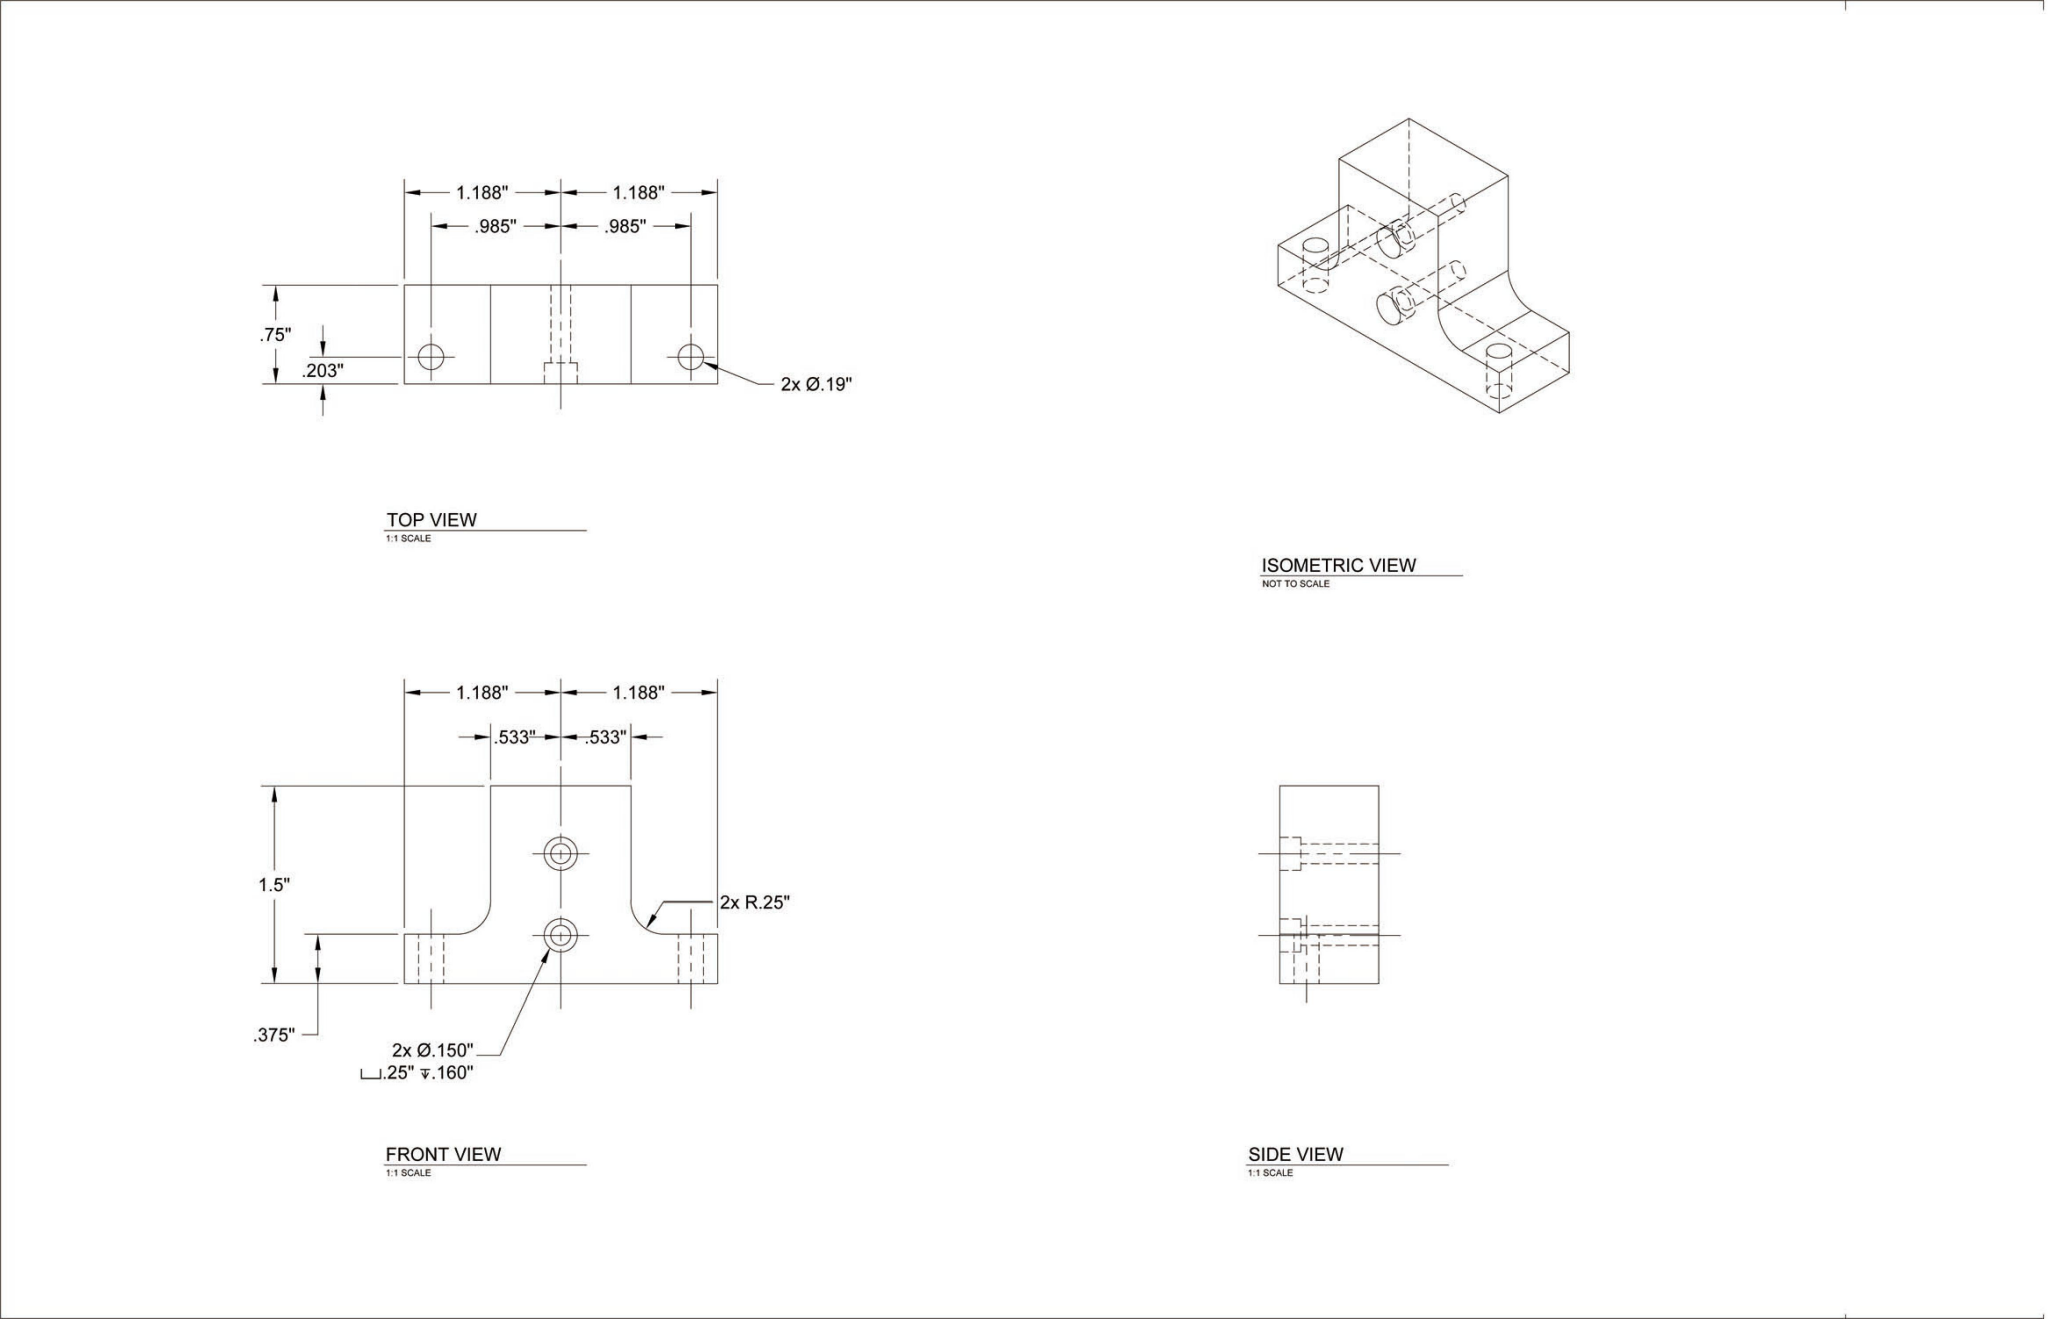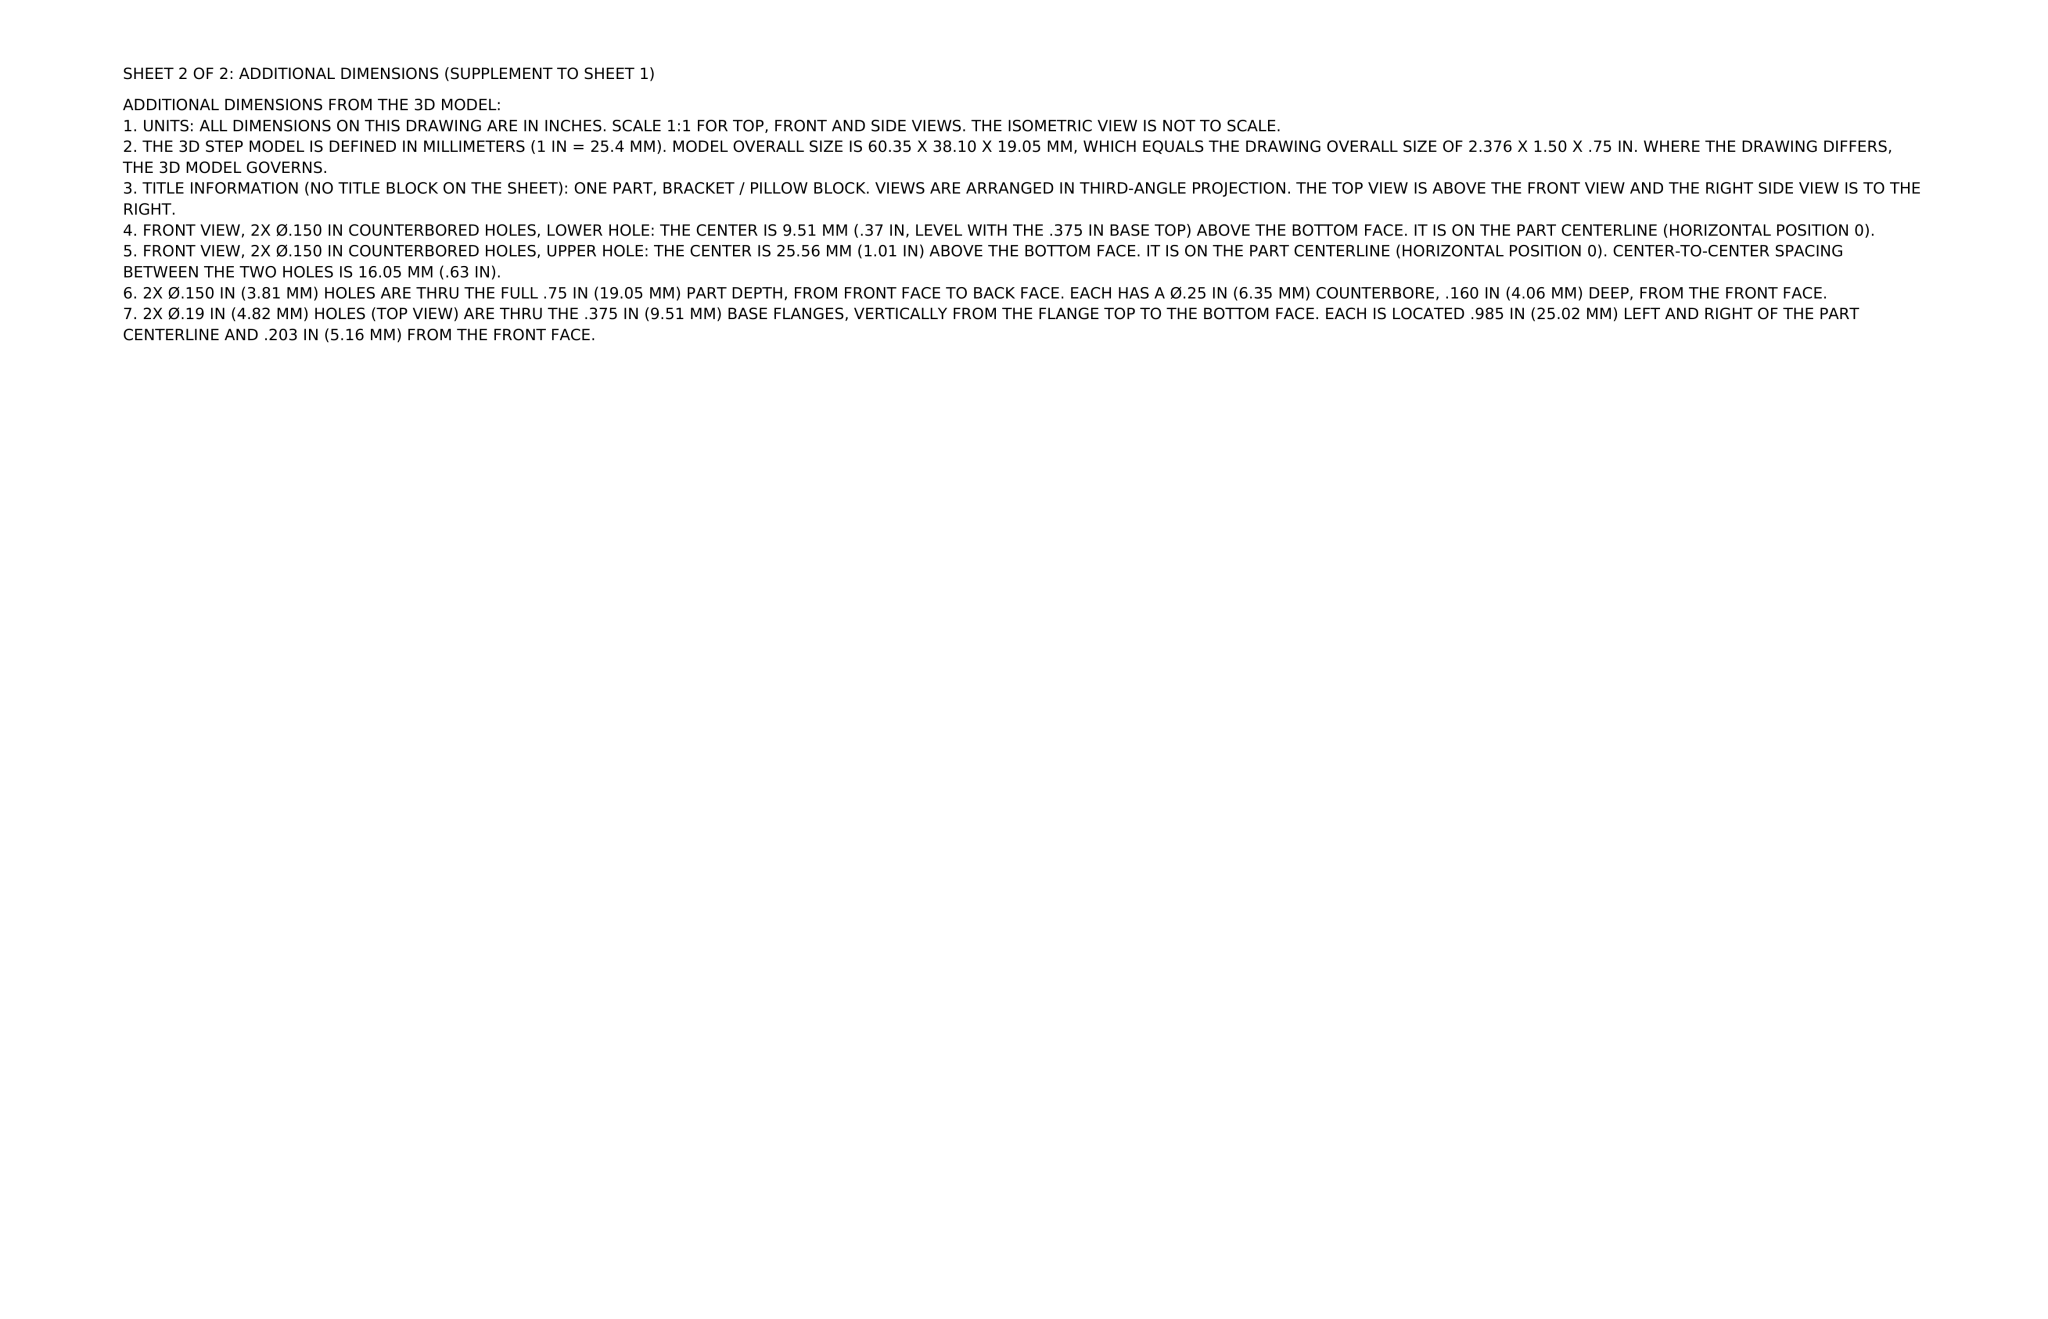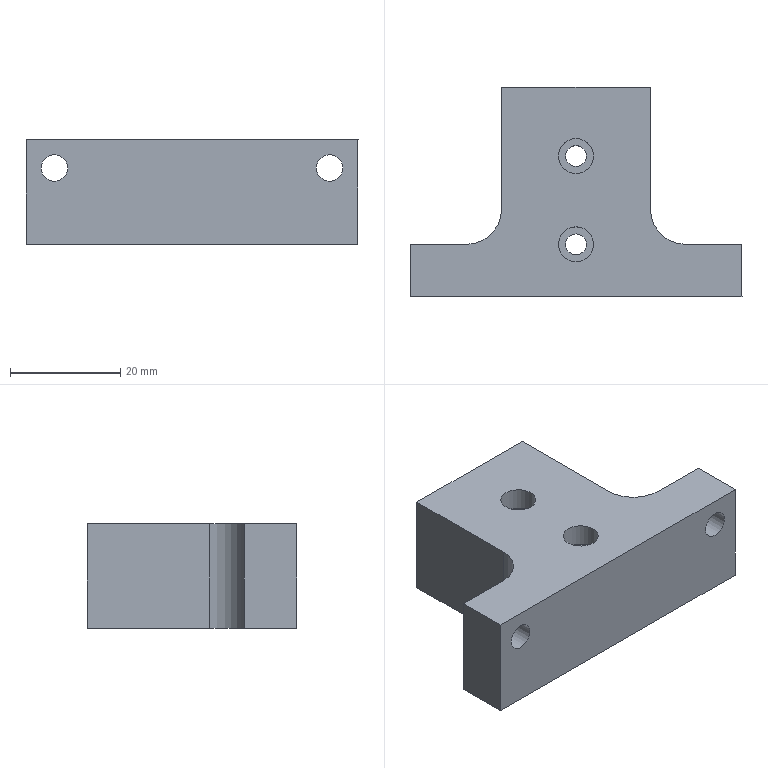Part | NX | mm | Notched Dual-Pedestal Mounting Block | 1 solid | 20 faces | box 60.35 x 38.1 x 19.06 mm | volume 25073 mm3 | plane 12 | cylinder 8 | commonest cylinder face diameters 3.81 x2 6.35 x2 4.82 x2 12.7 x2